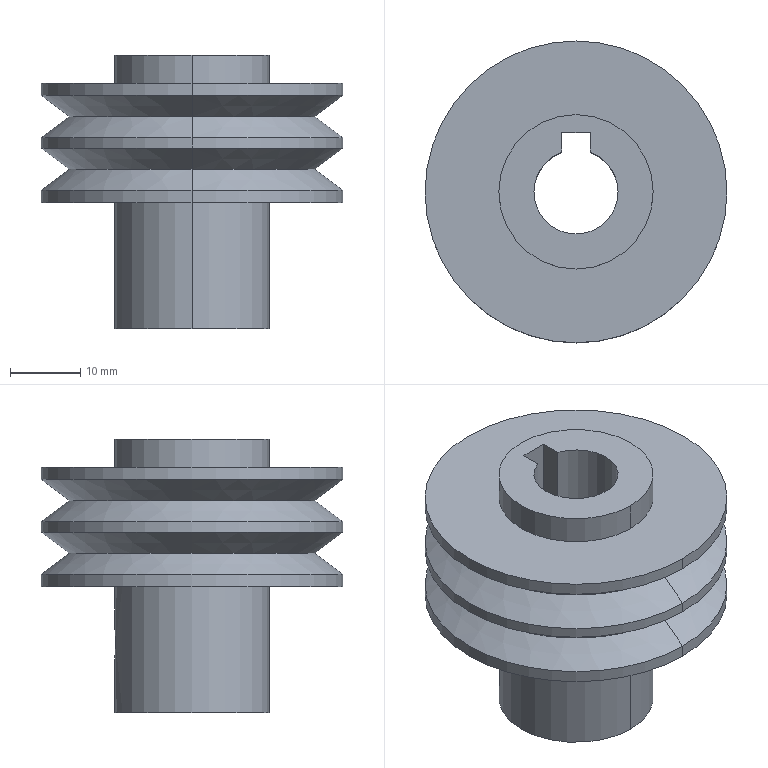Component | SolidWorks | SmallPulley-1 | 1 solid | 29 faces | box 43 x 43 x 39 mm | volume 25157 mm3 | cylinder 13 | cone 8 | plane 8 | commonest cylinder face diameters 43 x6 22 x4 4.2 x2 12 x1
build123d program:
from build123d import *

# Parameters (mm, degrees)
SKETCH2_W      = 4
SKETCH2_H      = 3
EXTRUDE1_DEPTH = 50.452


with BuildPart() as part:
    # Sketch1 → Revolve1 (revolve)
    with BuildSketch(Plane.XY, mode=Mode.PRIVATE) as revolve1_sk:
        Polygon((6, 47.92), (11, 47.92), (11, 43.92), (21.5, 43.92), (21.5, 42.17), (17.5, 39.17), (21.5, 36.17), (21.5, 34.67), (17.5, 31.67), (21.5, 28.67), (21.5, 26.92), (11, 26.92), (11, 8.92), (6, 8.92), align=None)
    revolve(revolve1_sk.sketch.rotate(Axis((0, 0, 0), (0, 1, 0)), 90), axis=Axis((0, 0, 0), (0, 1, 0)))

    # Sketch2 → Extrude1 (cut, through all)
    with BuildSketch(Plane(origin=(0, 47.92, 0), x_dir=(1, 0, 0), z_dir=(0, 1, 0))):
        with Locations((0, 7)):
            Rectangle(SKETCH2_W, SKETCH2_H)
    extrude(amount=-EXTRUDE1_DEPTH, mode=Mode.SUBTRACT)

    # Sketch3 → M5 Tapped Hole1 (revolve, cut)
    with BuildSketch(Plane(origin=(0.5139, 18.92, -8.5), x_dir=(0, -1, 0), z_dir=(1, 0, 0))):
        Polygon((0, 0), (0, 15.262), (2.1, 14), (2.1, 0), align=None)
    revolve(axis=Axis((0.5139, 18.92, -2.15), (0, 0, -1)), mode=Mode.SUBTRACT)


solid = part.part

# Placed as in the assembly
solid = solid.moved(Location((-210.944, 573.983, 228.868), (90, 0, 0)))
STEP:
#1=COLOUR_RGB('',0.7922,0.8196,0.9333);
#2=FILL_AREA_STYLE_COLOUR('',#1);
#3=FILL_AREA_STYLE('',(#2));
#4=SURFACE_STYLE_FILL_AREA(#3);
#5=SURFACE_SIDE_STYLE('',(#4));
#6=SURFACE_STYLE_USAGE(.BOTH.,#5);
#7=PRESENTATION_STYLE_ASSIGNMENT((#6));
#8=CARTESIAN_POINT('',(-8.305,23.031,9.675));
#9=VERTEX_POINT('',#8);
#10=CARTESIAN_POINT('',(-8.367,23.026,9.755));
#11=VERTEX_POINT('',#10);
#12=CARTESIAN_POINT('',(-8.305,23.031,9.675));
#13=CARTESIAN_POINT('',(-8.309,23.031,9.676));
#14=CARTESIAN_POINT('',(-8.314,23.031,9.678));
#15=CARTESIAN_POINT('',(-8.322,23.031,9.682));
#16=CARTESIAN_POINT('',(-8.326,23.03,9.684));
#17=CARTESIAN_POINT('',(-8.334,23.03,9.689));
#18=CARTESIAN_POINT('',(-8.337,23.03,9.692));
#19=CARTESIAN_POINT('',(-8.344,23.029,9.698));
#20=CARTESIAN_POINT('',(-8.347,23.029,9.701));
#21=CARTESIAN_POINT('',(-8.353,23.028,9.708));
#22=CARTESIAN_POINT('',(-8.355,23.028,9.712));
#23=CARTESIAN_POINT('',(-8.36,23.027,9.72));
#24=CARTESIAN_POINT('',(-8.361,23.027,9.724));
#25=CARTESIAN_POINT('',(-8.364,23.027,9.733));
#26=CARTESIAN_POINT('',(-8.365,23.027,9.737));
#27=CARTESIAN_POINT('',(-8.367,23.026,9.746));
#28=CARTESIAN_POINT('',(-8.367,23.026,9.751));
#29=CARTESIAN_POINT('',(-8.367,23.026,9.755));
#30=B_SPLINE_CURVE_WITH_KNOTS('',3,(#12,#13,#14,#15,#16,#17,#18,#19,#20,#21,#22,#23,#24,#25,#26,#27,#28,#29),.UNSPECIFIED.,.F.,.F.,(4,2,2,2,2,2,2,2,4),(0.007632,0.007979,0.008325,0.008671,0.009017,0.009363,0.009709,0.01006,0.0104),.UNSPECIFIED.);
#31=EDGE_CURVE('',#9,#11,#30,.T.);
#32=ORIENTED_EDGE('',*,*,#31,.T.);
#33=CARTESIAN_POINT('',(-8.367,22.932,9.755));
#34=VERTEX_POINT('',#33);
#35=CARTESIAN_POINT('',(-8.367,22.932,9.755));
#36=DIRECTION('',(0.,-1.,0.));
#37=VECTOR('',#36,39.37);
#38=LINE('',#35,#37);
#39=EDGE_CURVE('',#11,#34,#38,.T.);
#40=ORIENTED_EDGE('',*,*,#39,.T.);
#41=CARTESIAN_POINT('',(-8.226,22.932,9.697));
#42=VERTEX_POINT('',#41);
#43=CARTESIAN_POINT('',(-8.285,22.932,9.755));
#44=DIRECTION('',(0.,-1.,0.));
#45=DIRECTION('',(1.,0.,0.));
#46=AXIS2_PLACEMENT_3D('',#43,#44,#45);
#47=CIRCLE('',#46,0.08268);
#48=EDGE_CURVE('',#34,#42,#47,.T.);
#49=ORIENTED_EDGE('',*,*,#48,.T.);
#50=CARTESIAN_POINT('',(-8.202,22.932,9.755));
#51=VERTEX_POINT('',#50);
#52=CARTESIAN_POINT('',(-8.285,22.932,9.755));
#53=DIRECTION('',(0.,-1.,0.));
#54=DIRECTION('',(1.,0.,0.));
#55=AXIS2_PLACEMENT_3D('',#52,#53,#54);
#56=CIRCLE('',#55,0.08268);
#57=EDGE_CURVE('',#42,#51,#56,.T.);
#58=ORIENTED_EDGE('',*,*,#57,.T.);
#59=CARTESIAN_POINT('',(-8.202,23.018,9.755));
#60=VERTEX_POINT('',#59);
#61=CARTESIAN_POINT('',(-8.202,22.932,9.755));
#62=DIRECTION('',(0.,-1.,0.));
#63=VECTOR('',#62,39.37);
#64=LINE('',#61,#63);
#65=EDGE_CURVE('',#60,#51,#64,.T.);
#66=ORIENTED_EDGE('',*,*,#65,.F.);
#67=CARTESIAN_POINT('',(-8.202,23.018,9.755));
#68=CARTESIAN_POINT('',(-8.202,23.018,9.749));
#69=CARTESIAN_POINT('',(-8.203,23.019,9.743));
#70=CARTESIAN_POINT('',(-8.206,23.019,9.731));
#71=CARTESIAN_POINT('',(-8.208,23.02,9.725));
#72=CARTESIAN_POINT('',(-8.216,23.022,9.708));
#73=CARTESIAN_POINT('',(-8.224,23.023,9.698));
#74=CARTESIAN_POINT('',(-8.239,23.026,9.686));
#75=CARTESIAN_POINT('',(-8.244,23.027,9.683));
#76=CARTESIAN_POINT('',(-8.255,23.028,9.678));
#77=CARTESIAN_POINT('',(-8.261,23.029,9.676));
#78=CARTESIAN_POINT('',(-8.274,23.03,9.673));
#79=CARTESIAN_POINT('',(-8.28,23.03,9.673));
#80=CARTESIAN_POINT('',(-8.293,23.031,9.673));
#81=CARTESIAN_POINT('',(-8.299,23.031,9.674));
#82=CARTESIAN_POINT('',(-8.305,23.031,9.675));
#83=B_SPLINE_CURVE_WITH_KNOTS('',3,(#67,#68,#69,#70,#71,#72,#73,#74,#75,#76,#77,#78,#79,#80,#81,#82),.UNSPECIFIED.,.F.,.F.,(4,2,2,2,2,2,2,4),(0.003816,0.004293,0.00477,0.005724,0.006201,0.006678,0.007155,0.007632),.UNSPECIFIED.);
#84=EDGE_CURVE('',#60,#9,#83,.T.);
#85=ORIENTED_EDGE('',*,*,#84,.T.);
#86=EDGE_LOOP('',(#32,#40,#49,#58,#66,#85));
#87=FACE_OUTER_BOUND('',#86,.T.);
#88=CARTESIAN_POINT('',(-8.285,22.932,9.755));
#89=DIRECTION('',(0.,-1.,0.));
#90=DIRECTION('',(1.,0.,0.));
#91=AXIS2_PLACEMENT_3D('',#88,#89,#90);
#92=CYLINDRICAL_SURFACE('',#91,0.08268);
#93=ADVANCED_FACE('',(#87),#92,.F.);
#94=CARTESIAN_POINT('',(-8.305,23.031,10.07));
#95=VERTEX_POINT('',#94);
#96=CARTESIAN_POINT('',(-8.305,22.165,10.07));
#97=VERTEX_POINT('',#96);
#98=CARTESIAN_POINT('',(-8.305,22.598,10.07));
#99=DIRECTION('',(0.,0.,-1.));
#100=DIRECTION('',(0.,1.,0.));
#101=AXIS2_PLACEMENT_3D('',#98,#99,#100);
#102=CIRCLE('',#101,0.4331);
#103=EDGE_CURVE('',#95,#97,#102,.T.);
#104=ORIENTED_EDGE('',*,*,#103,.T.);
#105=CARTESIAN_POINT('',(-8.305,22.165,9.362));
#106=VERTEX_POINT('',#105);
#107=CARTESIAN_POINT('',(-8.305,22.165,9.011));
#108=DIRECTION('',(0.,0.,-1.));
#109=VECTOR('',#108,39.37);
#110=LINE('',#107,#109);
#111=EDGE_CURVE('',#97,#106,#110,.T.);
#112=ORIENTED_EDGE('',*,*,#111,.T.);
#113=CARTESIAN_POINT('',(-8.305,23.031,9.362));
#114=VERTEX_POINT('',#113);
#115=CARTESIAN_POINT('',(-8.305,22.598,9.362));
#116=DIRECTION('',(0.,0.,-1.));
#117=DIRECTION('',(0.,1.,0.));
#118=AXIS2_PLACEMENT_3D('',#115,#116,#117);
#119=CIRCLE('',#118,0.4331);
#120=EDGE_CURVE('',#114,#106,#119,.T.);
#121=ORIENTED_EDGE('',*,*,#120,.F.);
#122=CARTESIAN_POINT('',(-8.305,23.031,9.011));
#123=DIRECTION('',(0.,0.,-1.));
#124=VECTOR('',#123,39.37);
#125=LINE('',#122,#124);
#126=EDGE_CURVE('',#9,#114,#125,.T.);
#127=ORIENTED_EDGE('',*,*,#126,.F.);
#128=ORIENTED_EDGE('',*,*,#84,.F.);
#129=CARTESIAN_POINT('',(-8.305,23.031,9.836));
#130=VERTEX_POINT('',#129);
#131=CARTESIAN_POINT('',(-8.305,23.031,9.836));
#132=CARTESIAN_POINT('',(-8.299,23.031,9.837));
#133=CARTESIAN_POINT('',(-8.292,23.031,9.838));
#134=CARTESIAN_POINT('',(-8.28,23.03,9.838));
#135=CARTESIAN_POINT('',(-8.274,23.03,9.838));
#136=CARTESIAN_POINT('',(-8.255,23.028,9.834));
#137=CARTESIAN_POINT('',(-8.244,23.027,9.828));
#138=CARTESIAN_POINT('',(-8.229,23.024,9.817));
#139=CARTESIAN_POINT('',(-8.224,23.023,9.812));
#140=CARTESIAN_POINT('',(-8.217,23.022,9.803));
#141=CARTESIAN_POINT('',(-8.213,23.021,9.797));
#142=CARTESIAN_POINT('',(-8.208,23.02,9.786));
#143=CARTESIAN_POINT('',(-8.206,23.019,9.78));
#144=CARTESIAN_POINT('',(-8.203,23.019,9.768));
#145=CARTESIAN_POINT('',(-8.202,23.018,9.762));
#146=CARTESIAN_POINT('',(-8.202,23.018,9.755));
#147=B_SPLINE_CURVE_WITH_KNOTS('',3,(#131,#132,#133,#134,#135,#136,#137,#138,#139,#140,#141,#142,#143,#144,#145,#146),.UNSPECIFIED.,.F.,.F.,(4,2,2,2,2,2,2,4),(0.,0.000477,0.0009539,0.001908,0.002385,0.002862,0.003339,0.003816),.UNSPECIFIED.);
#148=EDGE_CURVE('',#130,#60,#147,.T.);
#149=ORIENTED_EDGE('',*,*,#148,.F.);
#150=CARTESIAN_POINT('',(-8.305,23.031,9.011));
#151=DIRECTION('',(0.,0.,-1.));
#152=VECTOR('',#151,39.37);
#153=LINE('',#150,#152);
#154=EDGE_CURVE('',#95,#130,#153,.T.);
#155=ORIENTED_EDGE('',*,*,#154,.F.);
#156=EDGE_LOOP('',(#104,#112,#121,#127,#128,#149,#155));
#157=FACE_OUTER_BOUND('',#156,.T.);
#158=CARTESIAN_POINT('',(-8.305,22.598,9.011));
#159=DIRECTION('',(0.,0.,-1.));
#160=DIRECTION('',(0.,1.,0.));
#161=AXIS2_PLACEMENT_3D('',#158,#159,#160);
#162=CYLINDRICAL_SURFACE('',#161,0.4331);
#163=ADVANCED_FACE('',(#157),#162,.T.);
#164=CARTESIAN_POINT('',(-8.305,23.444,10.139));
#165=VERTEX_POINT('',#164);
#166=CARTESIAN_POINT('',(-8.305,21.751,10.139));
#167=VERTEX_POINT('',#166);
#168=CARTESIAN_POINT('',(-8.305,22.598,10.139));
#169=DIRECTION('',(0.,0.,-1.));
#170=DIRECTION('',(0.,1.,0.));
#171=AXIS2_PLACEMENT_3D('',#168,#169,#170);
#172=CIRCLE('',#171,0.8465);
#173=EDGE_CURVE('',#165,#167,#172,.T.);
#174=ORIENTED_EDGE('',*,*,#173,.T.);
#175=CARTESIAN_POINT('',(-8.305,21.751,10.07));
#176=VERTEX_POINT('',#175);
#177=CARTESIAN_POINT('',(-8.305,21.751,9.011));
#178=DIRECTION('',(0.,0.,-1.));
#179=VECTOR('',#178,39.37);
#180=LINE('',#177,#179);
#181=EDGE_CURVE('',#167,#176,#180,.T.);
#182=ORIENTED_EDGE('',*,*,#181,.T.);
#183=CARTESIAN_POINT('',(-8.305,23.444,10.07));
#184=VERTEX_POINT('',#183);
#185=CARTESIAN_POINT('',(-8.305,22.598,10.07));
#186=DIRECTION('',(0.,0.,-1.));
#187=DIRECTION('',(0.,1.,0.));
#188=AXIS2_PLACEMENT_3D('',#185,#186,#187);
#189=CIRCLE('',#188,0.8465);
#190=EDGE_CURVE('',#184,#176,#189,.T.);
#191=ORIENTED_EDGE('',*,*,#190,.F.);
#192=CARTESIAN_POINT('',(-8.305,23.444,9.011));
#193=DIRECTION('',(0.,0.,-1.));
#194=VECTOR('',#193,39.37);
#195=LINE('',#192,#194);
#196=EDGE_CURVE('',#165,#184,#195,.T.);
#197=ORIENTED_EDGE('',*,*,#196,.F.);
#198=EDGE_LOOP('',(#174,#182,#191,#197));
#199=FACE_OUTER_BOUND('',#198,.T.);
#200=CARTESIAN_POINT('',(-8.305,22.598,9.011));
#201=DIRECTION('',(0.,0.,-1.));
#202=DIRECTION('',(0.,1.,0.));
#203=AXIS2_PLACEMENT_3D('',#200,#201,#202);
#204=CYLINDRICAL_SURFACE('',#203,0.8465);
#205=ADVANCED_FACE('',(#199),#204,.T.);
#206=CARTESIAN_POINT('',(-8.305,23.287,10.257));
#207=VERTEX_POINT('',#206);
#208=CARTESIAN_POINT('',(-8.305,21.909,10.257));
#209=VERTEX_POINT('',#208);
#210=CARTESIAN_POINT('',(-8.305,22.598,10.257));
#211=DIRECTION('',(0.,0.,-1.));
#212=DIRECTION('',(0.,1.,0.));
#213=AXIS2_PLACEMENT_3D('',#210,#211,#212);
#214=CIRCLE('',#213,0.689);
#215=EDGE_CURVE('',#207,#209,#214,.T.);
#216=ORIENTED_EDGE('',*,*,#215,.T.);
#217=CARTESIAN_POINT('',(-8.305,21.751,10.139));
#218=DIRECTION('',(0.,-0.8,-0.6));
#219=VECTOR('',#218,39.37);
#220=LINE('',#217,#219);
#221=EDGE_CURVE('',#209,#167,#220,.T.);
#222=ORIENTED_EDGE('',*,*,#221,.T.);
#223=ORIENTED_EDGE('',*,*,#173,.F.);
#224=CARTESIAN_POINT('',(-8.305,23.444,10.139));
#225=DIRECTION('',(0.,0.8,-0.6));
#226=VECTOR('',#225,39.37);
#227=LINE('',#224,#226);
#228=EDGE_CURVE('',#207,#165,#227,.T.);
#229=ORIENTED_EDGE('',*,*,#228,.F.);
#230=EDGE_LOOP('',(#216,#222,#223,#229));
#231=FACE_OUTER_BOUND('',#230,.T.);
#232=CARTESIAN_POINT('',(-8.305,22.598,10.139));
#233=DIRECTION('',(0.,0.,-1.));
#234=DIRECTION('',(0.,1.,0.));
#235=AXIS2_PLACEMENT_3D('',#232,#233,#234);
#236=CONICAL_SURFACE('',#235,0.8465,0.9273);
#237=ADVANCED_FACE('',(#231),#236,.T.);
#238=ORIENTED_EDGE('',*,*,#215,.F.);
#239=CARTESIAN_POINT('',(-8.305,23.444,10.376));
#240=VERTEX_POINT('',#239);
#241=CARTESIAN_POINT('',(-8.305,23.287,10.257));
#242=DIRECTION('',(0.,0.8,0.6));
#243=VECTOR('',#242,39.37);
#244=LINE('',#241,#243);
#245=EDGE_CURVE('',#207,#240,#244,.T.);
#246=ORIENTED_EDGE('',*,*,#245,.T.);
#247=CARTESIAN_POINT('',(-8.305,21.751,10.376));
#248=VERTEX_POINT('',#247);
#249=CARTESIAN_POINT('',(-8.305,22.598,10.376));
#250=DIRECTION('',(0.,0.,-1.));
#251=DIRECTION('',(0.,1.,0.));
#252=AXIS2_PLACEMENT_3D('',#249,#250,#251);
#253=CIRCLE('',#252,0.8465);
#254=EDGE_CURVE('',#240,#248,#253,.T.);
#255=ORIENTED_EDGE('',*,*,#254,.T.);
#256=CARTESIAN_POINT('',(-8.305,21.909,10.257));
#257=DIRECTION('',(0.,-0.8,0.6));
#258=VECTOR('',#257,39.37);
#259=LINE('',#256,#258);
#260=EDGE_CURVE('',#209,#248,#259,.T.);
#261=ORIENTED_EDGE('',*,*,#260,.F.);
#262=EDGE_LOOP('',(#238,#246,#255,#261));
#263=FACE_OUTER_BOUND('',#262,.T.);
#264=CARTESIAN_POINT('',(-8.305,22.598,10.257));
#265=DIRECTION('',(0.,0.,1.));
#266=DIRECTION('',(0.,-1.,0.));
#267=AXIS2_PLACEMENT_3D('',#264,#265,#266);
#268=CONICAL_SURFACE('',#267,0.689,0.9273);
#269=ADVANCED_FACE('',(#263),#268,.T.);
#270=CARTESIAN_POINT('',(-8.305,23.444,10.435));
#271=VERTEX_POINT('',#270);
#272=CARTESIAN_POINT('',(-8.305,21.751,10.435));
#273=VERTEX_POINT('',#272);
#274=CARTESIAN_POINT('',(-8.305,22.598,10.435));
#275=DIRECTION('',(0.,0.,-1.));
#276=DIRECTION('',(0.,1.,0.));
#277=AXIS2_PLACEMENT_3D('',#274,#275,#276);
#278=CIRCLE('',#277,0.8465);
#279=EDGE_CURVE('',#271,#273,#278,.T.);
#280=ORIENTED_EDGE('',*,*,#279,.T.);
#281=CARTESIAN_POINT('',(-8.305,21.751,9.011));
#282=DIRECTION('',(0.,0.,-1.));
#283=VECTOR('',#282,39.37);
#284=LINE('',#281,#283);
#285=EDGE_CURVE('',#273,#248,#284,.T.);
#286=ORIENTED_EDGE('',*,*,#285,.T.);
#287=ORIENTED_EDGE('',*,*,#254,.F.);
#288=CARTESIAN_POINT('',(-8.305,23.444,9.011));
#289=DIRECTION('',(0.,0.,-1.));
#290=VECTOR('',#289,39.37);
#291=LINE('',#288,#290);
#292=EDGE_CURVE('',#271,#240,#291,.T.);
#293=ORIENTED_EDGE('',*,*,#292,.F.);
#294=EDGE_LOOP('',(#280,#286,#287,#293));
#295=FACE_OUTER_BOUND('',#294,.T.);
#296=CARTESIAN_POINT('',(-8.305,22.598,9.011));
#297=DIRECTION('',(0.,0.,-1.));
#298=DIRECTION('',(0.,1.,0.));
#299=AXIS2_PLACEMENT_3D('',#296,#297,#298);
#300=CYLINDRICAL_SURFACE('',#299,0.8465);
#301=ADVANCED_FACE('',(#295),#300,.T.);
#302=CARTESIAN_POINT('',(-8.305,23.287,10.553));
#303=VERTEX_POINT('',#302);
#304=CARTESIAN_POINT('',(-8.305,21.909,10.553));
#305=VERTEX_POINT('',#304);
#306=CARTESIAN_POINT('',(-8.305,22.598,10.553));
#307=DIRECTION('',(0.,0.,-1.));
#308=DIRECTION('',(0.,1.,0.));
#309=AXIS2_PLACEMENT_3D('',#306,#307,#308);
#310=CIRCLE('',#309,0.689);
#311=EDGE_CURVE('',#303,#305,#310,.T.);
#312=ORIENTED_EDGE('',*,*,#311,.T.);
#313=CARTESIAN_POINT('',(-8.305,21.751,10.435));
#314=DIRECTION('',(0.,-0.8,-0.6));
#315=VECTOR('',#314,39.37);
#316=LINE('',#313,#315);
#317=EDGE_CURVE('',#305,#273,#316,.T.);
#318=ORIENTED_EDGE('',*,*,#317,.T.);
#319=ORIENTED_EDGE('',*,*,#279,.F.);
#320=CARTESIAN_POINT('',(-8.305,23.444,10.435));
#321=DIRECTION('',(0.,0.8,-0.6));
#322=VECTOR('',#321,39.37);
#323=LINE('',#320,#322);
#324=EDGE_CURVE('',#303,#271,#323,.T.);
#325=ORIENTED_EDGE('',*,*,#324,.F.);
#326=EDGE_LOOP('',(#312,#318,#319,#325));
#327=FACE_OUTER_BOUND('',#326,.T.);
#328=CARTESIAN_POINT('',(-8.305,22.598,10.435));
#329=DIRECTION('',(0.,0.,-1.));
#330=DIRECTION('',(0.,1.,0.));
#331=AXIS2_PLACEMENT_3D('',#328,#329,#330);
#332=CONICAL_SURFACE('',#331,0.8465,0.9273);
#333=ADVANCED_FACE('',(#327),#332,.T.);
#334=ORIENTED_EDGE('',*,*,#311,.F.);
#335=CARTESIAN_POINT('',(-8.305,23.444,10.671));
#336=VERTEX_POINT('',#335);
#337=CARTESIAN_POINT('',(-8.305,23.287,10.553));
#338=DIRECTION('',(0.,0.8,0.6));
#339=VECTOR('',#338,39.37);
#340=LINE('',#337,#339);
#341=EDGE_CURVE('',#303,#336,#340,.T.);
#342=ORIENTED_EDGE('',*,*,#341,.T.);
#343=CARTESIAN_POINT('',(-8.305,21.751,10.671));
#344=VERTEX_POINT('',#343);
#345=CARTESIAN_POINT('',(-8.305,22.598,10.671));
#346=DIRECTION('',(0.,0.,-1.));
#347=DIRECTION('',(0.,1.,0.));
#348=AXIS2_PLACEMENT_3D('',#345,#346,#347);
#349=CIRCLE('',#348,0.8465);
#350=EDGE_CURVE('',#336,#344,#349,.T.);
#351=ORIENTED_EDGE('',*,*,#350,.T.);
#352=CARTESIAN_POINT('',(-8.305,21.909,10.553));
#353=DIRECTION('',(0.,-0.8,0.6));
#354=VECTOR('',#353,39.37);
#355=LINE('',#352,#354);
#356=EDGE_CURVE('',#305,#344,#355,.T.);
#357=ORIENTED_EDGE('',*,*,#356,.F.);
#358=EDGE_LOOP('',(#334,#342,#351,#357));
#359=FACE_OUTER_BOUND('',#358,.T.);
#360=CARTESIAN_POINT('',(-8.305,22.598,10.553));
#361=DIRECTION('',(0.,0.,1.));
#362=DIRECTION('',(0.,-1.,0.));
#363=AXIS2_PLACEMENT_3D('',#360,#361,#362);
#364=CONICAL_SURFACE('',#363,0.689,0.9273);
#365=ADVANCED_FACE('',(#359),#364,.T.);
#366=CARTESIAN_POINT('',(-8.305,23.444,10.74));
#367=VERTEX_POINT('',#366);
#368=CARTESIAN_POINT('',(-8.305,21.751,10.74));
#369=VERTEX_POINT('',#368);
#370=CARTESIAN_POINT('',(-8.305,22.598,10.74));
#371=DIRECTION('',(0.,0.,-1.));
#372=DIRECTION('',(0.,1.,0.));
#373=AXIS2_PLACEMENT_3D('',#370,#371,#372);
#374=CIRCLE('',#373,0.8465);
#375=EDGE_CURVE('',#367,#369,#374,.T.);
#376=ORIENTED_EDGE('',*,*,#375,.T.);
#377=CARTESIAN_POINT('',(-8.305,21.751,9.011));
#378=DIRECTION('',(0.,0.,-1.));
#379=VECTOR('',#378,39.37);
#380=LINE('',#377,#379);
#381=EDGE_CURVE('',#369,#344,#380,.T.);
#382=ORIENTED_EDGE('',*,*,#381,.T.);
#383=ORIENTED_EDGE('',*,*,#350,.F.);
#384=CARTESIAN_POINT('',(-8.305,23.444,9.011));
#385=DIRECTION('',(0.,0.,-1.));
#386=VECTOR('',#385,39.37);
#387=LINE('',#384,#386);
#388=EDGE_CURVE('',#367,#336,#387,.T.);
#389=ORIENTED_EDGE('',*,*,#388,.F.);
#390=EDGE_LOOP('',(#376,#382,#383,#389));
#391=FACE_OUTER_BOUND('',#390,.T.);
#392=CARTESIAN_POINT('',(-8.305,22.598,9.011));
#393=DIRECTION('',(0.,0.,-1.));
#394=DIRECTION('',(0.,1.,0.));
#395=AXIS2_PLACEMENT_3D('',#392,#393,#394);
#396=CYLINDRICAL_SURFACE('',#395,0.8465);
#397=ADVANCED_FACE('',(#391),#396,.T.);
#398=CARTESIAN_POINT('',(-8.305,23.031,10.897));
#399=VERTEX_POINT('',#398);
#400=CARTESIAN_POINT('',(-8.305,22.165,10.897));
#401=VERTEX_POINT('',#400);
#402=CARTESIAN_POINT('',(-8.305,22.598,10.897));
#403=DIRECTION('',(0.,0.,-1.));
#404=DIRECTION('',(0.,1.,0.));
#405=AXIS2_PLACEMENT_3D('',#402,#403,#404);
#406=CIRCLE('',#405,0.4331);
#407=EDGE_CURVE('',#399,#401,#406,.T.);
#408=ORIENTED_EDGE('',*,*,#407,.T.);
#409=CARTESIAN_POINT('',(-8.305,22.165,10.74));
#410=VERTEX_POINT('',#409);
#411=CARTESIAN_POINT('',(-8.305,22.165,9.011));
#412=DIRECTION('',(0.,0.,-1.));
#413=VECTOR('',#412,39.37);
#414=LINE('',#411,#413);
#415=EDGE_CURVE('',#401,#410,#414,.T.);
#416=ORIENTED_EDGE('',*,*,#415,.T.);
#417=CARTESIAN_POINT('',(-8.305,23.031,10.74));
#418=VERTEX_POINT('',#417);
#419=CARTESIAN_POINT('',(-8.305,22.598,10.74));
#420=DIRECTION('',(0.,0.,-1.));
#421=DIRECTION('',(0.,1.,0.));
#422=AXIS2_PLACEMENT_3D('',#419,#420,#421);
#423=CIRCLE('',#422,0.4331);
#424=EDGE_CURVE('',#418,#410,#423,.T.);
#425=ORIENTED_EDGE('',*,*,#424,.F.);
#426=CARTESIAN_POINT('',(-8.305,23.031,9.011));
#427=DIRECTION('',(0.,0.,-1.));
#428=VECTOR('',#427,39.37);
#429=LINE('',#426,#428);
#430=EDGE_CURVE('',#399,#418,#429,.T.);
#431=ORIENTED_EDGE('',*,*,#430,.F.);
#432=EDGE_LOOP('',(#408,#416,#425,#431));
#433=FACE_OUTER_BOUND('',#432,.T.);
#434=CARTESIAN_POINT('',(-8.305,22.598,9.011));
#435=DIRECTION('',(0.,0.,-1.));
#436=DIRECTION('',(0.,1.,0.));
#437=AXIS2_PLACEMENT_3D('',#434,#435,#436);
#438=CYLINDRICAL_SURFACE('',#437,0.4331);
#439=ADVANCED_FACE('',(#433),#438,.T.);
#440=CARTESIAN_POINT('',(-8.384,22.82,10.897));
#441=VERTEX_POINT('',#440);
#442=CARTESIAN_POINT('',(-8.384,22.82,9.362));
#443=VERTEX_POINT('',#442);
#444=CARTESIAN_POINT('',(-8.384,22.82,9.011));
#445=DIRECTION('',(0.,0.,-1.));
#446=VECTOR('',#445,39.37);
#447=LINE('',#444,#446);
#448=EDGE_CURVE('',#441,#443,#447,.T.);
#449=ORIENTED_EDGE('',*,*,#448,.F.);
#450=CARTESIAN_POINT('',(-8.226,22.82,10.897));
#451=VERTEX_POINT('',#450);
#452=CARTESIAN_POINT('',(-8.305,22.598,10.897));
#453=DIRECTION('',(0.,0.,-1.));
#454=DIRECTION('',(0.,1.,0.));
#455=AXIS2_PLACEMENT_3D('',#452,#453,#454);
#456=CIRCLE('',#455,0.2362);
#457=EDGE_CURVE('',#451,#441,#456,.T.);
#458=ORIENTED_EDGE('',*,*,#457,.F.);
#459=CARTESIAN_POINT('',(-8.226,22.82,9.362));
#460=VERTEX_POINT('',#459);
#461=CARTESIAN_POINT('',(-8.226,22.82,9.011));
#462=DIRECTION('',(0.,0.,1.));
#463=VECTOR('',#462,39.37);
#464=LINE('',#461,#463);
#465=EDGE_CURVE('',#460,#451,#464,.T.);
#466=ORIENTED_EDGE('',*,*,#465,.F.);
#467=CARTESIAN_POINT('',(-8.305,22.598,9.362));
#468=DIRECTION('',(0.,0.,-1.));
#469=DIRECTION('',(0.,1.,0.));
#470=AXIS2_PLACEMENT_3D('',#467,#468,#469);
#471=CIRCLE('',#470,0.2362);
#472=EDGE_CURVE('',#460,#443,#471,.T.);
#473=ORIENTED_EDGE('',*,*,#472,.T.);
#474=EDGE_LOOP('',(#449,#458,#466,#473));
#475=FACE_OUTER_BOUND('',#474,.T.);
#476=CARTESIAN_POINT('',(-8.305,22.598,9.011));
#477=DIRECTION('',(0.,0.,-1.));
#478=DIRECTION('',(0.,1.,0.));
#479=AXIS2_PLACEMENT_3D('',#476,#477,#478);
#480=CYLINDRICAL_SURFACE('',#479,0.2362);
#481=ADVANCED_FACE('',(#475),#480,.F.);
#482=CARTESIAN_POINT('',(-8.384,22.932,10.897));
#483=VERTEX_POINT('',#482);
#484=CARTESIAN_POINT('',(-8.384,22.932,10.897));
#485=DIRECTION('',(0.,-1.,0.));
#486=VECTOR('',#485,39.37);
#487=LINE('',#484,#486);
#488=EDGE_CURVE('',#483,#441,#487,.T.);
#489=ORIENTED_EDGE('',*,*,#488,.F.);
#490=CARTESIAN_POINT('',(-8.226,22.932,10.897));
#491=VERTEX_POINT('',#490);
#492=CARTESIAN_POINT('',(-8.384,22.932,10.897));
#493=DIRECTION('',(-1.,0.,0.));
#494=VECTOR('',#493,39.37);
#495=LINE('',#492,#494);
#496=EDGE_CURVE('',#491,#483,#495,.T.);
#497=ORIENTED_EDGE('',*,*,#496,.F.);
#498=CARTESIAN_POINT('',(-8.226,22.932,10.897));
#499=DIRECTION('',(-0.,1.,0.));
#500=VECTOR('',#499,39.37);
#501=LINE('',#498,#500);
#502=EDGE_CURVE('',#451,#491,#501,.T.);
#503=ORIENTED_EDGE('',*,*,#502,.F.);
#504=ORIENTED_EDGE('',*,*,#457,.T.);
#505=EDGE_LOOP('',(#489,#497,#503,#504));
#506=FACE_BOUND('',#505,.T.);
#507=ORIENTED_EDGE('',*,*,#407,.F.);
#508=CARTESIAN_POINT('',(-8.305,22.598,10.897));
#509=DIRECTION('',(0.,0.,-1.));
#510=DIRECTION('',(0.,1.,0.));
#511=AXIS2_PLACEMENT_3D('',#508,#509,#510);
#512=CIRCLE('',#511,0.4331);
#513=EDGE_CURVE('',#401,#399,#512,.T.);
#514=ORIENTED_EDGE('',*,*,#513,.F.);
#515=EDGE_LOOP('',(#507,#514));
#516=FACE_OUTER_BOUND('',#515,.T.);
#517=CARTESIAN_POINT('',(-8.069,22.598,10.897));
#518=DIRECTION('',(0.,0.,1.));
#519=DIRECTION('',(0.,-1.,0.));
#520=AXIS2_PLACEMENT_3D('',#517,#518,#519);
#521=PLANE('',#520);
#522=ADVANCED_FACE('',(#506,#516),#521,.T.);
#523=ORIENTED_EDGE('',*,*,#415,.F.);
#524=ORIENTED_EDGE('',*,*,#513,.T.);
#525=ORIENTED_EDGE('',*,*,#430,.T.);
#526=CARTESIAN_POINT('',(-8.305,22.598,10.74));
#527=DIRECTION('',(0.,0.,-1.));
#528=DIRECTION('',(0.,1.,0.));
#529=AXIS2_PLACEMENT_3D('',#526,#527,#528);
#530=CIRCLE('',#529,0.4331);
#531=EDGE_CURVE('',#410,#418,#530,.T.);
#532=ORIENTED_EDGE('',*,*,#531,.F.);
#533=EDGE_LOOP('',(#523,#524,#525,#532));
#534=FACE_OUTER_BOUND('',#533,.T.);
#535=CARTESIAN_POINT('',(-8.305,22.598,9.011));
#536=DIRECTION('',(0.,0.,-1.));
#537=DIRECTION('',(0.,1.,0.));
#538=AXIS2_PLACEMENT_3D('',#535,#536,#537);
#539=CYLINDRICAL_SURFACE('',#538,0.4331);
#540=ADVANCED_FACE('',(#534),#539,.T.);
#541=ORIENTED_EDGE('',*,*,#424,.T.);
#542=ORIENTED_EDGE('',*,*,#531,.T.);
#543=EDGE_LOOP('',(#541,#542));
#544=FACE_BOUND('',#543,.T.);
#545=ORIENTED_EDGE('',*,*,#375,.F.);
#546=CARTESIAN_POINT('',(-8.305,22.598,10.74));
#547=DIRECTION('',(0.,0.,-1.));
#548=DIRECTION('',(0.,1.,0.));
#549=AXIS2_PLACEMENT_3D('',#546,#547,#548);
#550=CIRCLE('',#549,0.8465);
#551=EDGE_CURVE('',#369,#367,#550,.T.);
#552=ORIENTED_EDGE('',*,*,#551,.F.);
#553=EDGE_LOOP('',(#545,#552));
#554=FACE_OUTER_BOUND('',#553,.T.);
#555=CARTESIAN_POINT('',(-7.872,22.598,10.74));
#556=DIRECTION('',(0.,0.,1.));
#557=DIRECTION('',(0.,-1.,0.));
#558=AXIS2_PLACEMENT_3D('',#555,#556,#557);
#559=PLANE('',#558);
#560=ADVANCED_FACE('',(#544,#554),#559,.T.);
#561=ORIENTED_EDGE('',*,*,#381,.F.);
#562=ORIENTED_EDGE('',*,*,#551,.T.);
#563=ORIENTED_EDGE('',*,*,#388,.T.);
#564=CARTESIAN_POINT('',(-8.305,22.598,10.671));
#565=DIRECTION('',(0.,0.,-1.));
#566=DIRECTION('',(0.,1.,0.));
#567=AXIS2_PLACEMENT_3D('',#564,#565,#566);
#568=CIRCLE('',#567,0.8465);
#569=EDGE_CURVE('',#344,#336,#568,.T.);
#570=ORIENTED_EDGE('',*,*,#569,.F.);
#571=EDGE_LOOP('',(#561,#562,#563,#570));
#572=FACE_OUTER_BOUND('',#571,.T.);
#573=CARTESIAN_POINT('',(-8.305,22.598,9.011));
#574=DIRECTION('',(0.,0.,-1.));
#575=DIRECTION('',(0.,1.,0.));
#576=AXIS2_PLACEMENT_3D('',#573,#574,#575);
#577=CYLINDRICAL_SURFACE('',#576,0.8465);
#578=ADVANCED_FACE('',(#572),#577,.T.);
#579=ORIENTED_EDGE('',*,*,#341,.F.);
#580=CARTESIAN_POINT('',(-8.305,22.598,10.553));
#581=DIRECTION('',(0.,0.,-1.));
#582=DIRECTION('',(0.,1.,0.));
#583=AXIS2_PLACEMENT_3D('',#580,#581,#582);
#584=CIRCLE('',#583,0.689);
#585=EDGE_CURVE('',#305,#303,#584,.T.);
#586=ORIENTED_EDGE('',*,*,#585,.F.);
#587=ORIENTED_EDGE('',*,*,#356,.T.);
#588=ORIENTED_EDGE('',*,*,#569,.T.);
#589=EDGE_LOOP('',(#579,#586,#587,#588));
#590=FACE_OUTER_BOUND('',#589,.T.);
#591=CARTESIAN_POINT('',(-8.305,22.598,10.553));
#592=DIRECTION('',(0.,0.,1.));
#593=DIRECTION('',(0.,-1.,0.));
#594=AXIS2_PLACEMENT_3D('',#591,#592,#593);
#595=CONICAL_SURFACE('',#594,0.689,0.9273);
#596=ADVANCED_FACE('',(#590),#595,.T.);
#597=ORIENTED_EDGE('',*,*,#317,.F.);
#598=ORIENTED_EDGE('',*,*,#585,.T.);
#599=ORIENTED_EDGE('',*,*,#324,.T.);
#600=CARTESIAN_POINT('',(-8.305,22.598,10.435));
#601=DIRECTION('',(0.,0.,-1.));
#602=DIRECTION('',(0.,1.,0.));
#603=AXIS2_PLACEMENT_3D('',#600,#601,#602);
#604=CIRCLE('',#603,0.8465);
#605=EDGE_CURVE('',#273,#271,#604,.T.);
#606=ORIENTED_EDGE('',*,*,#605,.F.);
#607=EDGE_LOOP('',(#597,#598,#599,#606));
#608=FACE_OUTER_BOUND('',#607,.T.);
#609=CARTESIAN_POINT('',(-8.305,22.598,10.435));
#610=DIRECTION('',(0.,0.,-1.));
#611=DIRECTION('',(0.,1.,0.));
#612=AXIS2_PLACEMENT_3D('',#609,#610,#611);
#613=CONICAL_SURFACE('',#612,0.8465,0.9273);
#614=ADVANCED_FACE('',(#608),#613,.T.);
#615=ORIENTED_EDGE('',*,*,#285,.F.);
#616=ORIENTED_EDGE('',*,*,#605,.T.);
#617=ORIENTED_EDGE('',*,*,#292,.T.);
#618=CARTESIAN_POINT('',(-8.305,22.598,10.376));
#619=DIRECTION('',(0.,0.,-1.));
#620=DIRECTION('',(0.,1.,0.));
#621=AXIS2_PLACEMENT_3D('',#618,#619,#620);
#622=CIRCLE('',#621,0.8465);
#623=EDGE_CURVE('',#248,#240,#622,.T.);
#624=ORIENTED_EDGE('',*,*,#623,.F.);
#625=EDGE_LOOP('',(#615,#616,#617,#624));
#626=FACE_OUTER_BOUND('',#625,.T.);
#627=CARTESIAN_POINT('',(-8.305,22.598,9.011));
#628=DIRECTION('',(0.,0.,-1.));
#629=DIRECTION('',(0.,1.,0.));
#630=AXIS2_PLACEMENT_3D('',#627,#628,#629);
#631=CYLINDRICAL_SURFACE('',#630,0.8465);
#632=ADVANCED_FACE('',(#626),#631,.T.);
#633=ORIENTED_EDGE('',*,*,#245,.F.);
#634=CARTESIAN_POINT('',(-8.305,22.598,10.257));
#635=DIRECTION('',(0.,0.,-1.));
#636=DIRECTION('',(0.,1.,0.));
#637=AXIS2_PLACEMENT_3D('',#634,#635,#636);
#638=CIRCLE('',#637,0.689);
#639=EDGE_CURVE('',#209,#207,#638,.T.);
#640=ORIENTED_EDGE('',*,*,#639,.F.);
#641=ORIENTED_EDGE('',*,*,#260,.T.);
#642=ORIENTED_EDGE('',*,*,#623,.T.);
#643=EDGE_LOOP('',(#633,#640,#641,#642));
#644=FACE_OUTER_BOUND('',#643,.T.);
#645=CARTESIAN_POINT('',(-8.305,22.598,10.257));
#646=DIRECTION('',(0.,0.,1.));
#647=DIRECTION('',(0.,-1.,0.));
#648=AXIS2_PLACEMENT_3D('',#645,#646,#647);
#649=CONICAL_SURFACE('',#648,0.689,0.9273);
#650=ADVANCED_FACE('',(#644),#649,.T.);
#651=ORIENTED_EDGE('',*,*,#221,.F.);
#652=ORIENTED_EDGE('',*,*,#639,.T.);
#653=ORIENTED_EDGE('',*,*,#228,.T.);
#654=CARTESIAN_POINT('',(-8.305,22.598,10.139));
#655=DIRECTION('',(0.,0.,-1.));
#656=DIRECTION('',(0.,1.,0.));
#657=AXIS2_PLACEMENT_3D('',#654,#655,#656);
#658=CIRCLE('',#657,0.8465);
#659=EDGE_CURVE('',#167,#165,#658,.T.);
#660=ORIENTED_EDGE('',*,*,#659,.F.);
#661=EDGE_LOOP('',(#651,#652,#653,#660));
#662=FACE_OUTER_BOUND('',#661,.T.);
#663=CARTESIAN_POINT('',(-8.305,22.598,10.139));
#664=DIRECTION('',(0.,0.,-1.));
#665=DIRECTION('',(0.,1.,0.));
#666=AXIS2_PLACEMENT_3D('',#663,#664,#665);
#667=CONICAL_SURFACE('',#666,0.8465,0.9273);
#668=ADVANCED_FACE('',(#662),#667,.T.);
#669=ORIENTED_EDGE('',*,*,#181,.F.);
#670=ORIENTED_EDGE('',*,*,#659,.T.);
#671=ORIENTED_EDGE('',*,*,#196,.T.);
#672=CARTESIAN_POINT('',(-8.305,22.598,10.07));
#673=DIRECTION('',(0.,0.,-1.));
#674=DIRECTION('',(0.,1.,0.));
#675=AXIS2_PLACEMENT_3D('',#672,#673,#674);
#676=CIRCLE('',#675,0.8465);
#677=EDGE_CURVE('',#176,#184,#676,.T.);
#678=ORIENTED_EDGE('',*,*,#677,.F.);
#679=EDGE_LOOP('',(#669,#670,#671,#678));
#680=FACE_OUTER_BOUND('',#679,.T.);
#681=CARTESIAN_POINT('',(-8.305,22.598,9.011));
#682=DIRECTION('',(0.,0.,-1.));
#683=DIRECTION('',(0.,1.,0.));
#684=AXIS2_PLACEMENT_3D('',#681,#682,#683);
#685=CYLINDRICAL_SURFACE('',#684,0.8465);
#686=ADVANCED_FACE('',(#680),#685,.T.);
#687=ORIENTED_EDGE('',*,*,#190,.T.);
#688=ORIENTED_EDGE('',*,*,#677,.T.);
#689=EDGE_LOOP('',(#687,#688));
#690=FACE_OUTER_BOUND('',#689,.T.);
#691=ORIENTED_EDGE('',*,*,#103,.F.);
#692=CARTESIAN_POINT('',(-8.305,22.598,10.07));
#693=DIRECTION('',(0.,0.,-1.));
#694=DIRECTION('',(0.,1.,0.));
#695=AXIS2_PLACEMENT_3D('',#692,#693,#694);
#696=CIRCLE('',#695,0.4331);
#697=EDGE_CURVE('',#97,#95,#696,.T.);
#698=ORIENTED_EDGE('',*,*,#697,.F.);
#699=EDGE_LOOP('',(#691,#698));
#700=FACE_BOUND('',#699,.T.);
#701=CARTESIAN_POINT('',(-7.458,22.598,10.07));
#702=DIRECTION('',(0.,0.,-1.));
#703=DIRECTION('',(0.,1.,0.));
#704=AXIS2_PLACEMENT_3D('',#701,#702,#703);
#705=PLANE('',#704);
#706=ADVANCED_FACE('',(#690,#700),#705,.T.);
#707=ORIENTED_EDGE('',*,*,#111,.F.);
#708=ORIENTED_EDGE('',*,*,#697,.T.);
#709=ORIENTED_EDGE('',*,*,#154,.T.);
#710=CARTESIAN_POINT('',(-8.367,23.026,9.755));
#711=CARTESIAN_POINT('',(-8.367,23.026,9.76));
#712=CARTESIAN_POINT('',(-8.367,23.026,9.765));
#713=CARTESIAN_POINT('',(-8.365,23.027,9.774));
#714=CARTESIAN_POINT('',(-8.364,23.027,9.778));
#715=CARTESIAN_POINT('',(-8.361,23.027,9.787));
#716=CARTESIAN_POINT('',(-8.359,23.027,9.791));
#717=CARTESIAN_POINT('',(-8.355,23.028,9.799));
#718=CARTESIAN_POINT('',(-8.353,23.028,9.803));
#719=CARTESIAN_POINT('',(-8.347,23.029,9.81));
#720=CARTESIAN_POINT('',(-8.344,23.029,9.813));
#721=CARTESIAN_POINT('',(-8.337,23.03,9.819));
#722=CARTESIAN_POINT('',(-8.334,23.03,9.822));
#723=CARTESIAN_POINT('',(-8.326,23.03,9.827));
#724=CARTESIAN_POINT('',(-8.322,23.031,9.829));
#725=CARTESIAN_POINT('',(-8.314,23.031,9.833));
#726=CARTESIAN_POINT('',(-8.309,23.031,9.834));
#727=CARTESIAN_POINT('',(-8.305,23.031,9.836));
#728=B_SPLINE_CURVE_WITH_KNOTS('',3,(#710,#711,#712,#713,#714,#715,#716,#717,#718,#719,#720,#721,#722,#723,#724,#725,#726,#727),.UNSPECIFIED.,.F.,.F.,(4,2,2,2,2,2,2,2,4),(0.0104,0.01075,0.01109,0.01144,0.01178,0.01213,0.01248,0.01282,0.01317),.UNSPECIFIED.);
#729=EDGE_CURVE('',#11,#130,#728,.T.);
#730=ORIENTED_EDGE('',*,*,#729,.F.);
#731=ORIENTED_EDGE('',*,*,#31,.F.);
#732=ORIENTED_EDGE('',*,*,#126,.T.);
#733=CARTESIAN_POINT('',(-8.305,22.598,9.362));
#734=DIRECTION('',(0.,0.,-1.));
#735=DIRECTION('',(0.,1.,0.));
#736=AXIS2_PLACEMENT_3D('',#733,#734,#735);
#737=CIRCLE('',#736,0.4331);
#738=EDGE_CURVE('',#106,#114,#737,.T.);
#739=ORIENTED_EDGE('',*,*,#738,.F.);
#740=EDGE_LOOP('',(#707,#708,#709,#730,#731,#732,#739));
#741=FACE_OUTER_BOUND('',#740,.T.);
#742=CARTESIAN_POINT('',(-8.305,22.598,9.011));
#743=DIRECTION('',(0.,0.,-1.));
#744=DIRECTION('',(0.,1.,0.));
#745=AXIS2_PLACEMENT_3D('',#742,#743,#744);
#746=CYLINDRICAL_SURFACE('',#745,0.4331);
#747=ADVANCED_FACE('',(#741),#746,.T.);
#748=CARTESIAN_POINT('',(-8.384,22.932,9.362));
#749=VERTEX_POINT('',#748);
#750=CARTESIAN_POINT('',(-8.384,22.932,9.362));
#751=DIRECTION('',(0.,-1.,0.));
#752=VECTOR('',#751,39.37);
#753=LINE('',#750,#752);
#754=EDGE_CURVE('',#749,#443,#753,.T.);
#755=ORIENTED_EDGE('',*,*,#754,.T.);
#756=ORIENTED_EDGE('',*,*,#472,.F.);
#757=CARTESIAN_POINT('',(-8.226,22.932,9.362));
#758=VERTEX_POINT('',#757);
#759=CARTESIAN_POINT('',(-8.226,22.598,9.362));
#760=DIRECTION('',(0.,-1.,0.));
#761=VECTOR('',#760,39.37);
#762=LINE('',#759,#761);
#763=EDGE_CURVE('',#758,#460,#762,.T.);
#764=ORIENTED_EDGE('',*,*,#763,.F.);
#765=CARTESIAN_POINT('',(-8.384,22.932,9.362));
#766=DIRECTION('',(-1.,0.,0.));
#767=VECTOR('',#766,39.37);
#768=LINE('',#765,#767);
#769=EDGE_CURVE('',#758,#749,#768,.T.);
#770=ORIENTED_EDGE('',*,*,#769,.T.);
#771=EDGE_LOOP('',(#755,#756,#764,#770));
#772=FACE_BOUND('',#771,.T.);
#773=ORIENTED_EDGE('',*,*,#120,.T.);
#774=ORIENTED_EDGE('',*,*,#738,.T.);
#775=EDGE_LOOP('',(#773,#774));
#776=FACE_OUTER_BOUND('',#775,.T.);
#777=CARTESIAN_POINT('',(-7.872,22.598,9.362));
#778=DIRECTION('',(0.,0.,-1.));
#779=DIRECTION('',(0.,1.,0.));
#780=AXIS2_PLACEMENT_3D('',#777,#778,#779);
#781=PLANE('',#780);
#782=ADVANCED_FACE('',(#772,#776),#781,.T.);
#783=ORIENTED_EDGE('',*,*,#448,.T.);
#784=ORIENTED_EDGE('',*,*,#754,.F.);
#785=CARTESIAN_POINT('',(-8.384,22.932,9.362));
#786=DIRECTION('',(0.,0.,1.));
#787=VECTOR('',#786,39.37);
#788=LINE('',#785,#787);
#789=EDGE_CURVE('',#749,#483,#788,.T.);
#790=ORIENTED_EDGE('',*,*,#789,.T.);
#791=ORIENTED_EDGE('',*,*,#488,.T.);
#792=EDGE_LOOP('',(#783,#784,#790,#791));
#793=FACE_OUTER_BOUND('',#792,.T.);
#794=CARTESIAN_POINT('',(-8.384,22.932,9.362));
#795=DIRECTION('',(-1.,-0.,0.));
#796=DIRECTION('',(0.,-1.,0.));
#797=AXIS2_PLACEMENT_3D('',#794,#795,#796);
#798=PLANE('',#797);
#799=ADVANCED_FACE('',(#793),#798,.F.);
#800=CARTESIAN_POINT('',(-8.226,22.932,9.362));
#801=DIRECTION('',(0.,0.,1.));
#802=VECTOR('',#801,39.37);
#803=LINE('',#800,#802);
#804=EDGE_CURVE('',#758,#42,#803,.T.);
#805=ORIENTED_EDGE('',*,*,#804,.T.);
#806=ORIENTED_EDGE('',*,*,#48,.F.);
#807=CARTESIAN_POINT('',(-8.226,22.932,9.814));
#808=VERTEX_POINT('',#807);
#809=CARTESIAN_POINT('',(-8.285,22.932,9.755));
#810=DIRECTION('',(0.,-1.,0.));
#811=DIRECTION('',(1.,0.,0.));
#812=AXIS2_PLACEMENT_3D('',#809,#810,#811);
#813=CIRCLE('',#812,0.08268);
#814=EDGE_CURVE('',#808,#34,#813,.T.);
#815=ORIENTED_EDGE('',*,*,#814,.F.);
#816=CARTESIAN_POINT('',(-8.226,22.932,9.362));
#817=DIRECTION('',(0.,0.,1.));
#818=VECTOR('',#817,39.37);
#819=LINE('',#816,#818);
#820=EDGE_CURVE('',#808,#491,#819,.T.);
#821=ORIENTED_EDGE('',*,*,#820,.T.);
#822=ORIENTED_EDGE('',*,*,#496,.T.);
#823=ORIENTED_EDGE('',*,*,#789,.F.);
#824=ORIENTED_EDGE('',*,*,#769,.F.);
#825=EDGE_LOOP('',(#805,#806,#815,#821,#822,#823,#824));
#826=FACE_OUTER_BOUND('',#825,.T.);
#827=CARTESIAN_POINT('',(-8.384,22.932,9.362));
#828=DIRECTION('',(0.,1.,0.));
#829=DIRECTION('',(-1.,0.,0.));
#830=AXIS2_PLACEMENT_3D('',#827,#828,#829);
#831=PLANE('',#830);
#832=ADVANCED_FACE('',(#826),#831,.F.);
#833=ORIENTED_EDGE('',*,*,#465,.T.);
#834=ORIENTED_EDGE('',*,*,#502,.T.);
#835=ORIENTED_EDGE('',*,*,#820,.F.);
#836=CARTESIAN_POINT('',(-8.226,22.932,9.362));
#837=DIRECTION('',(0.,0.,1.));
#838=VECTOR('',#837,39.37);
#839=LINE('',#836,#838);
#840=EDGE_CURVE('',#42,#808,#839,.T.);
#841=ORIENTED_EDGE('',*,*,#840,.F.);
#842=ORIENTED_EDGE('',*,*,#804,.F.);
#843=ORIENTED_EDGE('',*,*,#763,.T.);
#844=EDGE_LOOP('',(#833,#834,#835,#841,#842,#843));
#845=FACE_OUTER_BOUND('',#844,.T.);
#846=CARTESIAN_POINT('',(-8.226,22.932,9.362));
#847=DIRECTION('',(1.,0.,0.));
#848=DIRECTION('',(-0.,1.,0.));
#849=AXIS2_PLACEMENT_3D('',#846,#847,#848);
#850=PLANE('',#849);
#851=ADVANCED_FACE('',(#845),#850,.F.);
#852=ORIENTED_EDGE('',*,*,#57,.F.);
#853=ORIENTED_EDGE('',*,*,#840,.T.);
#854=CARTESIAN_POINT('',(-8.285,22.932,9.755));
#855=DIRECTION('',(0.,-1.,0.));
#856=DIRECTION('',(1.,0.,0.));
#857=AXIS2_PLACEMENT_3D('',#854,#855,#856);
#858=CIRCLE('',#857,0.08268);
#859=EDGE_CURVE('',#51,#808,#858,.T.);
#860=ORIENTED_EDGE('',*,*,#859,.F.);
#861=EDGE_LOOP('',(#852,#853,#860));
#862=FACE_OUTER_BOUND('',#861,.T.);
#863=CARTESIAN_POINT('',(-8.202,22.932,9.755));
#864=DIRECTION('',(0.,-1.,0.));
#865=DIRECTION('',(1.,0.,0.));
#866=AXIS2_PLACEMENT_3D('',#863,#864,#865);
#867=PLANE('',#866);
#868=ADVANCED_FACE('',(#862),#867,.F.);
#869=ORIENTED_EDGE('',*,*,#39,.F.);
#870=ORIENTED_EDGE('',*,*,#729,.T.);
#871=ORIENTED_EDGE('',*,*,#148,.T.);
#872=ORIENTED_EDGE('',*,*,#65,.T.);
#873=ORIENTED_EDGE('',*,*,#859,.T.);
#874=ORIENTED_EDGE('',*,*,#814,.T.);
#875=EDGE_LOOP('',(#869,#870,#871,#872,#873,#874));
#876=FACE_OUTER_BOUND('',#875,.T.);
#877=CARTESIAN_POINT('',(-8.285,22.932,9.755));
#878=DIRECTION('',(0.,-1.,0.));
#879=DIRECTION('',(1.,0.,0.));
#880=AXIS2_PLACEMENT_3D('',#877,#878,#879);
#881=CYLINDRICAL_SURFACE('',#880,0.08268);
#882=ADVANCED_FACE('',(#876),#881,.F.);
#883=CLOSED_SHELL('',(#93,#163,#205,#237,#269,#301,#333,#365,#397,#439,#481,#522,#540,#560,#578,#596,#614,#632,#650,#668,#686,#706,#747,#782,#799,#832,#851,#868,#882));
#884=MANIFOLD_SOLID_BREP('',#883);
#885=STYLED_ITEM('',(#7),#884);
#886=PRESENTATION_LAYER_ASSIGNMENT('','',(#885));
#887=CARTESIAN_POINT('',(0.,0.,0.));
#888=DIRECTION('',(0.,0.,1.));
#889=DIRECTION('',(1.,0.,0.));
#890=AXIS2_PLACEMENT_3D('',#887,#888,#889);
#891=(LENGTH_UNIT()NAMED_UNIT(*)SI_UNIT($,.METRE.));
#892=LENGTH_MEASURE_WITH_UNIT(LENGTH_MEASURE(0.0254),#891);
#893=DIMENSIONAL_EXPONENTS(1.,0.,0.,0.,0.,0.,0.);
#894=(CONVERSION_BASED_UNIT('',#892)LENGTH_UNIT()NAMED_UNIT(#893));
#895=UNCERTAINTY_MEASURE_WITH_UNIT(LENGTH_MEASURE(0.00001),#894,'','');
#896=(NAMED_UNIT(*)PLANE_ANGLE_UNIT()SI_UNIT($,.RADIAN.));
#897=(NAMED_UNIT(*)SI_UNIT($,.STERADIAN.)SOLID_ANGLE_UNIT());
#898=(GEOMETRIC_REPRESENTATION_CONTEXT(3)GLOBAL_UNCERTAINTY_ASSIGNED_CONTEXT((#895))GLOBAL_UNIT_ASSIGNED_CONTEXT((#894,#896,#897))REPRESENTATION_CONTEXT('',''));
#899=ADVANCED_BREP_SHAPE_REPRESENTATION('',(#884,#890),#898);
#900=(LENGTH_UNIT()NAMED_UNIT(*)SI_UNIT($,.METRE.));
#901=LENGTH_MEASURE_WITH_UNIT(LENGTH_MEASURE(0.0254),#900);
#902=DIMENSIONAL_EXPONENTS(1.,0.,0.,0.,0.,0.,0.);
#903=(CONVERSION_BASED_UNIT('',#901)LENGTH_UNIT()NAMED_UNIT(#902));
#904=UNCERTAINTY_MEASURE_WITH_UNIT(LENGTH_MEASURE(0.00001),#903,'','');
#905=(NAMED_UNIT(*)PLANE_ANGLE_UNIT()SI_UNIT($,.RADIAN.));
#906=(NAMED_UNIT(*)SI_UNIT($,.STERADIAN.)SOLID_ANGLE_UNIT());
#907=(GEOMETRIC_REPRESENTATION_CONTEXT(3)GLOBAL_UNCERTAINTY_ASSIGNED_CONTEXT((#904))GLOBAL_UNIT_ASSIGNED_CONTEXT((#903,#905,#906))REPRESENTATION_CONTEXT('',''));
#908=MECHANICAL_DESIGN_GEOMETRIC_PRESENTATION_REPRESENTATION('',(#885),#907);